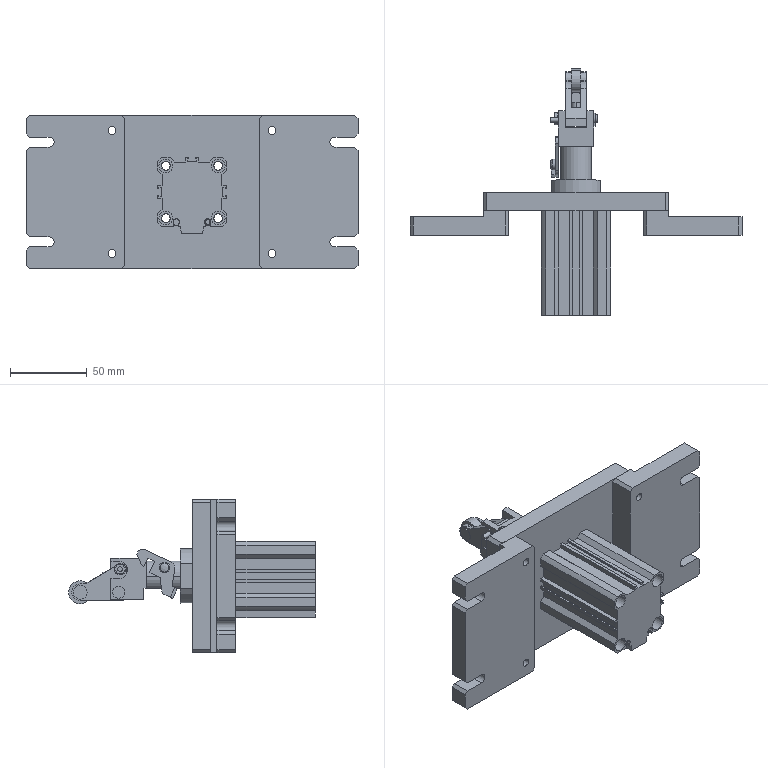Assembly | SolidWorks | mm | 9 component files | 9 solids | 421 faces | box 216 x 160.5 x 100 mm | volume 428860 mm3 | plane 239 | cylinder 155 | cone 24 | spline 3 | commonest cylinder face diameters 11 x22 9 x20 6.6 x16 5 x16 5.5 x8 4 x8 4.15 x6 6 x5
Bill of materials:
140507-L01M08U05-2-P01 | 1 |  | Flat rectangular plate with small corner chamfers, a large central through-hole, four small holes in a square pattern around it, and four corner through-holes.
140507-L01M08U05-2-P03(B) | 2 |  | Rectangular plate with chamfered corners, two through-holes near one long edge, and two open U-slots cut into the opposite edge. A raised step or lip runs along one end of the plate thickness.
RSDQ_D-M9BL_SW(32)_2 | 1 |  | Long stepped rod whose profile is a round section merged with a flat rectangular base or key along its length. A smaller round spigot sticks out from one end.
RSDQ_D-M9BL_SW(32) | 1 |  | Long stepped rod with a round section merged with a flat rectangular base along its length, and a smaller round spigot at the end opposite the one on unnamed part.
RSQ3220(0) | 1 |  | Flat profiled plate shaped roughly like an S or hook, with a rectangular notch near the upper end and a short round boss sticking out from one face. A small block-like step sits at the lower end.
RSQ32-20D(0)_ROD | 1 |  | Pin-like part made of a cylindrical shaft with a large flat disc head at one end and a square block at the other. The block has a slot through it, forming a clevis, and a small cross-pin passes through the slot.
RSQ32-20D_LEVER | 1 |  | Lever or bracket body: a roughly triangular block with a large rounded boss at one end and a through-hole at the other corner. It has a central window or slot holding a roller or cylinder, and a small stepped pin with a hex-like collar sticks out from one face.
RSQA32-20D(0)_BODY | 1 |  | Extruded square-profile body with chamfered corner lobes holding four through-holes, plus longitudinal T-slot-like grooves on its sides. A cylindrical boss or nose sticks out from one end.
Mates:
1. concentric | 140507-L01M08U05-2-P01-1 face at (-34.945, 10.344, -61.398) dir (0, 1, 0) r 5.5 | 140507-L01M08U05-2-P02-1 face at (-34.945, -1.656, -61.398) dir (0, 1, 0) r 2.5
2. concentric | 140507-L01M08U05-2-P01-1 face at (-34.945, 10.344, 18.602) dir (0, 1, 0) r 5.5 | 140507-L01M08U05-2-P02-1 face at (-34.945, -1.656, 18.602) dir (0, 1, 0) r 2.5
3. coincident | 140507-L01M08U05-2-P01-1 face at (17.055, -1.656, -21.398) dir (0, -1, 0) | 140507-L01M08U05-2-P02-1 face at (-40.945, -1.656, -71.398) dir (0, 1, 0)
4. concentric | 140507-L01M08U05-2-P01-1 face at (69.055, 10.344, 18.602) dir (0, 1, 0) r 5.5 | 140507-L01M08U05-2-P02-2 face at (69.055, -1.656, 18.602) dir (0, 1, 0) r 2.5
5. concentric | 140507-L01M08U05-2-P01-1 face at (69.055, 10.344, -61.398) dir (0, 1, 0) r 5.5 | 140507-L01M08U05-2-P02-2 face at (69.055, -1.656, -61.398) dir (0, 1, 0) r 2.5
6. coincident | 140507-L01M08U05-2-P01-1 face at (17.055, -1.656, -21.398) dir (0, -1, 0) | 140507-L01M08U05-2-P02-2 face at (75.055, -1.656, 28.602) dir (0, 1, 0)
7. concentric | 140507-L01M08U05-2-P02-1 face at (-34.945, -1.656, 18.602) dir (0, 1, 0) r 2.5 | 140507-L01M08U05-2-P03-1 face at (-34.945, -37.656, 18.602) dir (0, -1, 0) r 5.5
8. concentric | 140507-L01M08U05-2-P02-1 face at (-34.945, -1.656, -61.398) dir (0, 1, 0) r 2.5 | 140507-L01M08U05-2-P03-1 face at (-34.945, -37.656, -61.398) dir (0, -1, 0) r 5.5
9. coincident | 140507-L01M08U05-2-P02-1 face at (-40.945, -25.656, -71.398) dir (0, -1, 0) | 140507-L01M08U05-2-P03-1 face at (-58.945, -25.656, -21.398) dir (0, 1, 0)
10. concentric | 140507-L01M08U05-2-P02-2 face at (69.055, -1.656, 18.602) dir (0, 1, 0) r 2.5 | 140507-L01M08U05-2-P03-2 face at (69.055, -37.656, 18.602) dir (0, -1, 0) r 5.5
11. concentric | 140507-L01M08U05-2-P02-2 face at (69.055, -1.656, -61.398) dir (0, 1, 0) r 2.5 | 140507-L01M08U05-2-P03-2 face at (69.055, -37.656, -61.398) dir (0, -1, 0) r 5.5
12. coincident | 140507-L01M08U05-2-P02-2 face at (75.055, -25.656, 28.602) dir (0, -1, 0) | 140507-L01M08U05-2-P03-2 face at (93.055, -25.656, -21.398) dir (0, 1, 0)
13. coincident | 140507-L01M08U05-2-P01-1 face at (17.055, -1.656, -21.398) dir (0, -1, 0) | RSDQA32-20DD-M9BL(0_0)-1/RSQA32-20D(0)_BODY-1 face at (17.055, -1.656, -21.398) dir (0, 1, 0)
14. concentric | 140507-L01M08U05-2-P01-1 face at (17.055, -1.656, -21.398) dir (0, 1, 0) r 18.5 | RSDQA32-20DD-M9BL(0_0)-1/RSQA32-20D(0)_BODY-1 face at (17.055, 18.344, -21.398) dir (0, -1, 0) r 18
15. concentric | 140507-L01M08U05-2-P01-1 face at (34.055, 10.344, -38.398) dir (0, 1, 0) r 5.5 | RSDQA32-20DD-M9BL(0_0)-1/RSQA32-20D(0)_BODY-1 face at (34.055, -1.656, -38.398) dir (0, -1, 0) r 4.5
16. coincident | 140507-L01M08U05-2-P01-1 face at (17.055, -1.656, -21.398) dir (0, -1, 0) | 140507-L01M08U05-2-P03(B)-1 face at (93.055, -1.656, -21.398) dir (0, 1, 0)
17. concentric | 140507-L01M08U05-2-P01-1 face at (69.055, 10.344, -61.398) dir (0, 1, 0) r 3.3 | 140507-L01M08U05-2-P03(B)-1 face at (69.055, -1.656, -61.398) dir (0, 1, 0) r 2.5
18. concentric | 140507-L01M08U05-2-P01-1 face at (69.055, 10.344, 18.602) dir (0, 1, 0) r 3.3 | 140507-L01M08U05-2-P03(B)-1 face at (69.055, -1.656, 18.602) dir (0, 1, 0) r 2.5
19. coincident | 140507-L01M08U05-2-P01-1 face at (17.055, -1.656, -21.398) dir (0, -1, 0) | 140507-L01M08U05-2-P03(B)-2 face at (-58.945, -1.656, -21.398) dir (0, 1, 0)
20. concentric | 140507-L01M08U05-2-P01-1 face at (-34.945, 10.344, -61.398) dir (0, 1, 0) r 3.3 | 140507-L01M08U05-2-P03(B)-2 face at (-34.945, -1.656, -61.398) dir (0, 1, 0) r 2.5
21. concentric | 140507-L01M08U05-2-P01-1 face at (-34.945, 10.344, 18.602) dir (0, 1, 0) r 3.3 | 140507-L01M08U05-2-P03(B)-2 face at (-34.945, -1.656, 18.602) dir (0, 1, 0) r 2.5
22. distance | RSQA32-20D(0)_BODY-1 face at (-20, 0, 0) dir (-1, 0, 0) | RSQ32-20D(0)_ROD-1 face at (-42, -11.5, 11.5) dir (1, 0, 0)
23. concentric | RSQA32-20D(0)_BODY-1 face at (3.2, 0, 0) dir (-1, 0, 0) r 10 | RSQ32-20D(0)_ROD-1 face at (-7.8, 0, 0) dir (-1, 0, 0) r 10
24. parallel | RSQA32-20D(0)_BODY-1 face at (0, -11.2, 19.5) dir (0, 0, 1) | RSQ32-20D(0)_ROD-1 face at (-40, 0, 11.5) dir (0, 0, 1)
25. concentric | RSQ32-20D(0)_ROD-1 face at (-60, 10.5, 13.95) dir (0, 0, -1) r 2.5 | RSQ32-20D_LEVER-1 face at (-60, 10.5, 6.6) dir (0, 0, -1) r 2.5
26. width | RSQ32-20D(0)_ROD-1 face at (-40, 0, 7) dir (0, 0, -1) | RSQ32-20D(0)_ROD-1 face at (-40, 0, -7) dir (0, 0, 1) | RSQ32-20D_LEVER-1 face at (-60, 10.5, 6.6) dir (0, 0, 1) | RSQ32-20D_LEVER-1 face at (-60, 10.5, -6.6) dir (0, 0, -1)
27. coincident | RSQ32-20D(0)_ROD-1 face at (-40, 0, -11.5) dir (0, 0, -1) | RSQ3220(0)-1 face at (-21.131, 1.468, -11.5) dir (0, 0, 1)